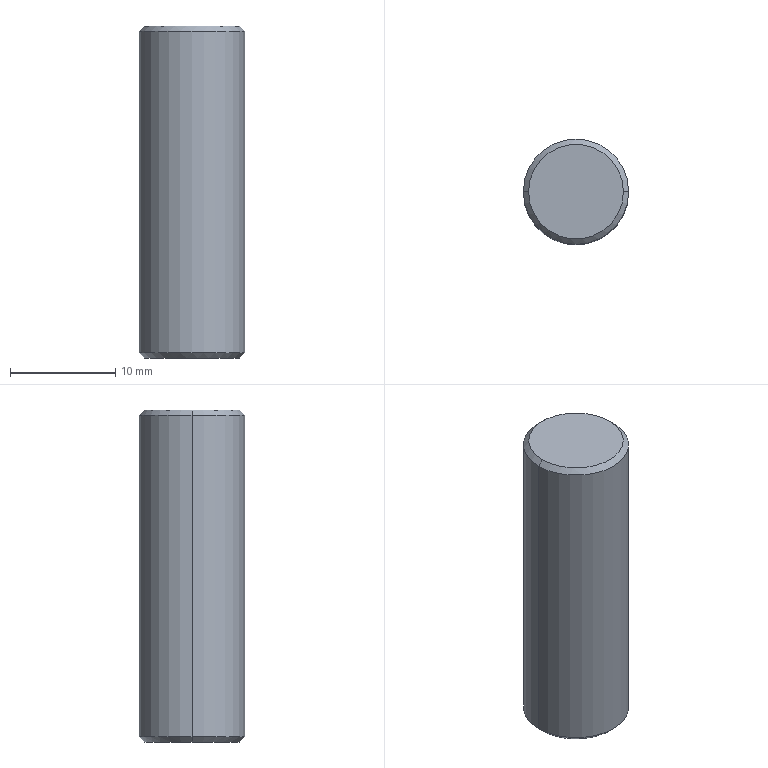Component | SolidWorks | ThreadedRodM10X30-1 | 1 solid | 8 faces | box 10 x 10 x 31.5 mm | volume 2466 mm3 | cone 4 | cylinder 2 | plane 2 | commonest cylinder face diameters 10 x2
build123d program:
from build123d import *

# Parameters (mm, degrees)
SKETCH1_W     = 31.5
SKETCH1_H     = 5
CHAMFER1_SIZE = 0.5


with BuildPart() as part:
    # Sketch1 → Revolve1 (revolve)
    with BuildSketch(Plane.XY, mode=Mode.PRIVATE) as revolve1_sk:
        with Locations((0, 2.5)):
            Rectangle(SKETCH1_W, SKETCH1_H)
    revolve(revolve1_sk.sketch.rotate(Axis((-60.119, 0, 0), (1, 0, 0)), 90), axis=Axis((-60.119, 0, 0), (1, 0, 0)))

    # Chamfer1
    chamfer1_edges = [part.edges().sort_by_distance(p)[0] for p in [
        (15.75, 0, -5),
        (-15.75, 0, -5),
    ]]
    chamfer(chamfer1_edges, length=CHAMFER1_SIZE)


solid = part.part

# Placed as in the assembly
solid = solid.moved(Location((7.266, 69.399, 36.75), (0, 90, 0)))
STEP:
#1=COLOUR_RGB('',0.7922,0.8196,0.9333);
#2=FILL_AREA_STYLE_COLOUR('',#1);
#3=FILL_AREA_STYLE('',(#2));
#4=SURFACE_STYLE_FILL_AREA(#3);
#5=SURFACE_SIDE_STYLE('',(#4));
#6=SURFACE_STYLE_USAGE(.BOTH.,#5);
#7=PRESENTATION_STYLE_ASSIGNMENT((#6));
#8=CARTESIAN_POINT('',(0.4632,2.732,2.067));
#9=VERTEX_POINT('',#8);
#10=CARTESIAN_POINT('',(0.1089,2.732,2.067));
#11=VERTEX_POINT('',#10);
#12=CARTESIAN_POINT('',(0.2861,2.732,2.067));
#13=DIRECTION('',(0.,0.,1.));
#14=DIRECTION('',(-1.,0.,0.));
#15=AXIS2_PLACEMENT_3D('',#12,#13,#14);
#16=CIRCLE('',#15,0.1772);
#17=EDGE_CURVE('',#9,#11,#16,.T.);
#18=ORIENTED_EDGE('',*,*,#17,.F.);
#19=CARTESIAN_POINT('',(0.4829,2.732,2.047));
#20=VERTEX_POINT('',#19);
#21=CARTESIAN_POINT('',(0.4632,2.732,2.067));
#22=DIRECTION('',(0.7071,0.,-0.7071));
#23=VECTOR('',#22,39.37);
#24=LINE('',#21,#23);
#25=EDGE_CURVE('',#9,#20,#24,.T.);
#26=ORIENTED_EDGE('',*,*,#25,.T.);
#27=CARTESIAN_POINT('',(0.08922,2.732,2.047));
#28=VERTEX_POINT('',#27);
#29=CARTESIAN_POINT('',(0.2861,2.732,2.047));
#30=DIRECTION('',(0.,0.,-1.));
#31=DIRECTION('',(-1.,0.,0.));
#32=AXIS2_PLACEMENT_3D('',#29,#30,#31);
#33=CIRCLE('',#32,0.1969);
#34=EDGE_CURVE('',#28,#20,#33,.T.);
#35=ORIENTED_EDGE('',*,*,#34,.F.);
#36=CARTESIAN_POINT('',(0.1089,2.732,2.067));
#37=DIRECTION('',(-0.7071,0.,-0.7071));
#38=VECTOR('',#37,39.37);
#39=LINE('',#36,#38);
#40=EDGE_CURVE('',#11,#28,#39,.T.);
#41=ORIENTED_EDGE('',*,*,#40,.F.);
#42=EDGE_LOOP('',(#18,#26,#35,#41));
#43=FACE_OUTER_BOUND('',#42,.T.);
#44=CARTESIAN_POINT('',(0.2861,2.732,2.067));
#45=DIRECTION('',(0.,0.,-1.));
#46=DIRECTION('',(-1.,0.,0.));
#47=AXIS2_PLACEMENT_3D('',#44,#45,#46);
#48=CONICAL_SURFACE('',#47,0.1772,0.7854);
#49=ADVANCED_FACE('',(#43),#48,.T.);
#50=CARTESIAN_POINT('',(0.1089,2.732,0.8268));
#51=VERTEX_POINT('',#50);
#52=CARTESIAN_POINT('',(0.4632,2.732,0.8268));
#53=VERTEX_POINT('',#52);
#54=CARTESIAN_POINT('',(0.2861,2.732,0.8268));
#55=DIRECTION('',(0.,0.,-1.));
#56=DIRECTION('',(1.,0.,0.));
#57=AXIS2_PLACEMENT_3D('',#54,#55,#56);
#58=CIRCLE('',#57,0.1772);
#59=EDGE_CURVE('',#51,#53,#58,.T.);
#60=ORIENTED_EDGE('',*,*,#59,.F.);
#61=CARTESIAN_POINT('',(0.08922,2.732,0.8465));
#62=VERTEX_POINT('',#61);
#63=CARTESIAN_POINT('',(0.08922,2.732,0.8465));
#64=DIRECTION('',(-0.7071,0.,0.7071));
#65=VECTOR('',#64,39.37);
#66=LINE('',#63,#65);
#67=EDGE_CURVE('',#51,#62,#66,.T.);
#68=ORIENTED_EDGE('',*,*,#67,.T.);
#69=CARTESIAN_POINT('',(0.4829,2.732,0.8465));
#70=VERTEX_POINT('',#69);
#71=CARTESIAN_POINT('',(0.2861,2.732,0.8465));
#72=DIRECTION('',(0.,0.,1.));
#73=DIRECTION('',(1.,0.,0.));
#74=AXIS2_PLACEMENT_3D('',#71,#72,#73);
#75=CIRCLE('',#74,0.1969);
#76=EDGE_CURVE('',#70,#62,#75,.T.);
#77=ORIENTED_EDGE('',*,*,#76,.F.);
#78=CARTESIAN_POINT('',(0.4829,2.732,0.8465));
#79=DIRECTION('',(0.7071,0.,0.7071));
#80=VECTOR('',#79,39.37);
#81=LINE('',#78,#80);
#82=EDGE_CURVE('',#53,#70,#81,.T.);
#83=ORIENTED_EDGE('',*,*,#82,.F.);
#84=EDGE_LOOP('',(#60,#68,#77,#83));
#85=FACE_OUTER_BOUND('',#84,.T.);
#86=CARTESIAN_POINT('',(0.2861,2.732,0.8465));
#87=DIRECTION('',(0.,0.,1.));
#88=DIRECTION('',(1.,0.,0.));
#89=AXIS2_PLACEMENT_3D('',#86,#87,#88);
#90=CONICAL_SURFACE('',#89,0.1969,0.7854);
#91=ADVANCED_FACE('',(#85),#90,.T.);
#92=ORIENTED_EDGE('',*,*,#76,.T.);
#93=CARTESIAN_POINT('',(0.08922,2.732,3.814));
#94=DIRECTION('',(0.,0.,1.));
#95=VECTOR('',#94,39.37);
#96=LINE('',#93,#95);
#97=EDGE_CURVE('',#62,#28,#96,.T.);
#98=ORIENTED_EDGE('',*,*,#97,.T.);
#99=ORIENTED_EDGE('',*,*,#34,.T.);
#100=CARTESIAN_POINT('',(0.4829,2.732,3.814));
#101=DIRECTION('',(0.,0.,1.));
#102=VECTOR('',#101,39.37);
#103=LINE('',#100,#102);
#104=EDGE_CURVE('',#70,#20,#103,.T.);
#105=ORIENTED_EDGE('',*,*,#104,.F.);
#106=EDGE_LOOP('',(#92,#98,#99,#105));
#107=FACE_OUTER_BOUND('',#106,.T.);
#108=CARTESIAN_POINT('',(0.2861,2.732,3.814));
#109=DIRECTION('',(0.,0.,1.));
#110=DIRECTION('',(1.,0.,0.));
#111=AXIS2_PLACEMENT_3D('',#108,#109,#110);
#112=CYLINDRICAL_SURFACE('',#111,0.1969);
#113=ADVANCED_FACE('',(#107),#112,.T.);
#114=CARTESIAN_POINT('',(0.2861,2.732,2.067));
#115=DIRECTION('',(0.,0.,1.));
#116=DIRECTION('',(-1.,0.,0.));
#117=AXIS2_PLACEMENT_3D('',#114,#115,#116);
#118=CIRCLE('',#117,0.1772);
#119=EDGE_CURVE('',#11,#9,#118,.T.);
#120=ORIENTED_EDGE('',*,*,#119,.T.);
#121=ORIENTED_EDGE('',*,*,#17,.T.);
#122=EDGE_LOOP('',(#120,#121));
#123=FACE_OUTER_BOUND('',#122,.T.);
#124=CARTESIAN_POINT('',(0.2861,2.732,2.067));
#125=DIRECTION('',(0.,0.,-1.));
#126=DIRECTION('',(-1.,0.,0.));
#127=AXIS2_PLACEMENT_3D('',#124,#125,#126);
#128=PLANE('',#127);
#129=ADVANCED_FACE('',(#123),#128,.F.);
#130=ORIENTED_EDGE('',*,*,#97,.F.);
#131=CARTESIAN_POINT('',(0.2861,2.732,0.8465));
#132=DIRECTION('',(0.,0.,1.));
#133=DIRECTION('',(1.,0.,0.));
#134=AXIS2_PLACEMENT_3D('',#131,#132,#133);
#135=CIRCLE('',#134,0.1969);
#136=EDGE_CURVE('',#62,#70,#135,.T.);
#137=ORIENTED_EDGE('',*,*,#136,.T.);
#138=ORIENTED_EDGE('',*,*,#104,.T.);
#139=CARTESIAN_POINT('',(0.2861,2.732,2.047));
#140=DIRECTION('',(0.,0.,-1.));
#141=DIRECTION('',(-1.,0.,0.));
#142=AXIS2_PLACEMENT_3D('',#139,#140,#141);
#143=CIRCLE('',#142,0.1969);
#144=EDGE_CURVE('',#20,#28,#143,.T.);
#145=ORIENTED_EDGE('',*,*,#144,.T.);
#146=EDGE_LOOP('',(#130,#137,#138,#145));
#147=FACE_OUTER_BOUND('',#146,.T.);
#148=CARTESIAN_POINT('',(0.2861,2.732,3.814));
#149=DIRECTION('',(0.,0.,1.));
#150=DIRECTION('',(1.,0.,0.));
#151=AXIS2_PLACEMENT_3D('',#148,#149,#150);
#152=CYLINDRICAL_SURFACE('',#151,0.1969);
#153=ADVANCED_FACE('',(#147),#152,.T.);
#154=CARTESIAN_POINT('',(0.2861,2.732,0.8268));
#155=DIRECTION('',(0.,0.,-1.));
#156=DIRECTION('',(1.,0.,0.));
#157=AXIS2_PLACEMENT_3D('',#154,#155,#156);
#158=CIRCLE('',#157,0.1772);
#159=EDGE_CURVE('',#53,#51,#158,.T.);
#160=ORIENTED_EDGE('',*,*,#159,.T.);
#161=ORIENTED_EDGE('',*,*,#59,.T.);
#162=EDGE_LOOP('',(#160,#161));
#163=FACE_OUTER_BOUND('',#162,.T.);
#164=CARTESIAN_POINT('',(0.2861,2.929,0.8268));
#165=DIRECTION('',(0.,0.,1.));
#166=DIRECTION('',(1.,0.,0.));
#167=AXIS2_PLACEMENT_3D('',#164,#165,#166);
#168=PLANE('',#167);
#169=ADVANCED_FACE('',(#163),#168,.F.);
#170=ORIENTED_EDGE('',*,*,#67,.F.);
#171=ORIENTED_EDGE('',*,*,#159,.F.);
#172=ORIENTED_EDGE('',*,*,#82,.T.);
#173=ORIENTED_EDGE('',*,*,#136,.F.);
#174=EDGE_LOOP('',(#170,#171,#172,#173));
#175=FACE_OUTER_BOUND('',#174,.T.);
#176=CARTESIAN_POINT('',(0.2861,2.732,0.8465));
#177=DIRECTION('',(0.,0.,1.));
#178=DIRECTION('',(1.,0.,0.));
#179=AXIS2_PLACEMENT_3D('',#176,#177,#178);
#180=CONICAL_SURFACE('',#179,0.1969,0.7854);
#181=ADVANCED_FACE('',(#175),#180,.T.);
#182=ORIENTED_EDGE('',*,*,#25,.F.);
#183=ORIENTED_EDGE('',*,*,#119,.F.);
#184=ORIENTED_EDGE('',*,*,#40,.T.);
#185=ORIENTED_EDGE('',*,*,#144,.F.);
#186=EDGE_LOOP('',(#182,#183,#184,#185));
#187=FACE_OUTER_BOUND('',#186,.T.);
#188=CARTESIAN_POINT('',(0.2861,2.732,2.067));
#189=DIRECTION('',(0.,0.,-1.));
#190=DIRECTION('',(-1.,0.,0.));
#191=AXIS2_PLACEMENT_3D('',#188,#189,#190);
#192=CONICAL_SURFACE('',#191,0.1772,0.7854);
#193=ADVANCED_FACE('',(#187),#192,.T.);
#194=CLOSED_SHELL('',(#49,#91,#113,#129,#153,#169,#181,#193));
#195=MANIFOLD_SOLID_BREP('',#194);
#196=STYLED_ITEM('',(#7),#195);
#197=(LENGTH_UNIT()NAMED_UNIT(*)SI_UNIT($,.METRE.));
#198=LENGTH_MEASURE_WITH_UNIT(LENGTH_MEASURE(0.0254),#197);
#199=DIMENSIONAL_EXPONENTS(1.,0.,0.,0.,0.,0.,0.);
#200=(CONVERSION_BASED_UNIT('',#198)LENGTH_UNIT()NAMED_UNIT(#199));
#201=UNCERTAINTY_MEASURE_WITH_UNIT(LENGTH_MEASURE(0.00001),#200,'','');
#202=(NAMED_UNIT(*)PLANE_ANGLE_UNIT()SI_UNIT($,.RADIAN.));
#203=(NAMED_UNIT(*)SI_UNIT($,.STERADIAN.)SOLID_ANGLE_UNIT());
#204=(GEOMETRIC_REPRESENTATION_CONTEXT(3)GLOBAL_UNCERTAINTY_ASSIGNED_CONTEXT((#201))GLOBAL_UNIT_ASSIGNED_CONTEXT((#200,#202,#203))REPRESENTATION_CONTEXT('',''));
#205=MECHANICAL_DESIGN_GEOMETRIC_PRESENTATION_REPRESENTATION('',(#196),#204);
#206=CARTESIAN_POINT('',(0.,0.,0.));
#207=DIRECTION('',(0.,0.,1.));
#208=DIRECTION('',(1.,0.,0.));
#209=AXIS2_PLACEMENT_3D('',#206,#207,#208);
#210=(LENGTH_UNIT()NAMED_UNIT(*)SI_UNIT($,.METRE.));
#211=LENGTH_MEASURE_WITH_UNIT(LENGTH_MEASURE(0.0254),#210);
#212=DIMENSIONAL_EXPONENTS(1.,0.,0.,0.,0.,0.,0.);
#213=(CONVERSION_BASED_UNIT('',#211)LENGTH_UNIT()NAMED_UNIT(#212));
#214=UNCERTAINTY_MEASURE_WITH_UNIT(LENGTH_MEASURE(0.00001),#213,'','');
#215=(NAMED_UNIT(*)PLANE_ANGLE_UNIT()SI_UNIT($,.RADIAN.));
#216=(NAMED_UNIT(*)SI_UNIT($,.STERADIAN.)SOLID_ANGLE_UNIT());
#217=(GEOMETRIC_REPRESENTATION_CONTEXT(3)GLOBAL_UNCERTAINTY_ASSIGNED_CONTEXT((#214))GLOBAL_UNIT_ASSIGNED_CONTEXT((#213,#215,#216))REPRESENTATION_CONTEXT('',''));
#218=ADVANCED_BREP_SHAPE_REPRESENTATION('',(#195,#209),#217);
#219=PRESENTATION_LAYER_ASSIGNMENT('','',(#196));